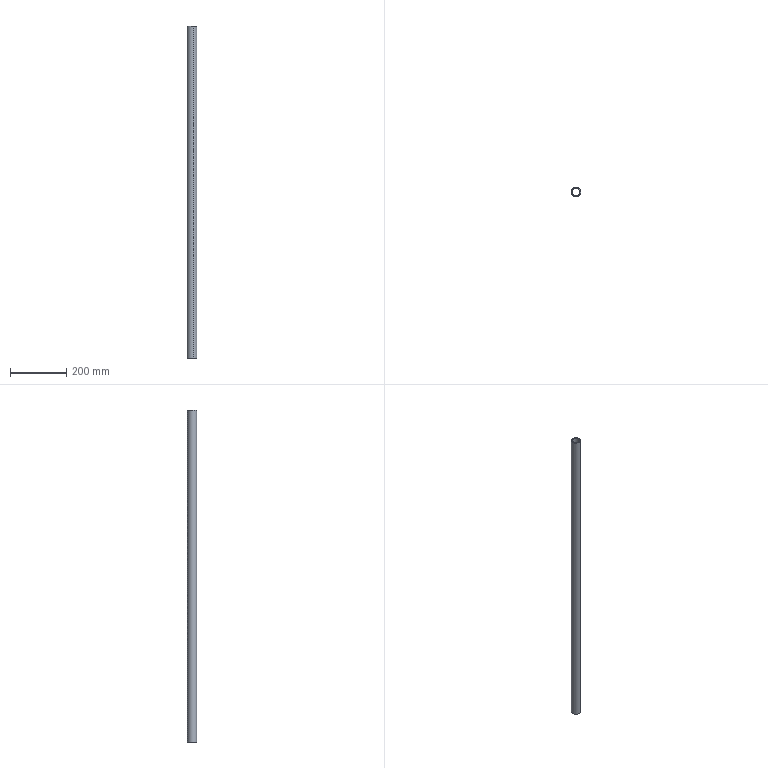Component | SolidWorks | PlatformGuardrail2-10 | 1 solid | 6 faces | box 33.5 x 33.5 x 1180 mm | volume 339198 mm3 | cylinder 4 | plane 2 | commonest cylinder face diameters 27.5 x2 33.5 x2 | material Plain Carbon Steel
build123d program:
from build123d import *

# Parameters (mm, degrees)
SKETCH1_R           = 16.75
SKETCH1_R_2         = 13.75
BOSS_EXTRUDE1_DEPTH = 1180


with BuildPart() as part:
    # Sketch1 → Boss-Extrude1 (new body)
    with BuildSketch(Plane(origin=(0, 0, 0), x_dir=(1, 0, 0), z_dir=(0, 1, 0))):
        with Locations(Location((0, 0, 0), (0, 0, 270))):
            Circle(SKETCH1_R)
        with Locations(Location((0, 0, 0), (0, 0, 270))):
            Circle(SKETCH1_R_2, mode=Mode.SUBTRACT)
    extrude(amount=BOSS_EXTRUDE1_DEPTH)


solid = part.part

# Placed as in the assembly
solid = solid.moved(Location((271.551, 2924.573, 5594.223), (90, 0, 0)))
STEP:
#1=COLOUR_RGB('',0.7922,0.8196,0.9333);
#2=FILL_AREA_STYLE_COLOUR('',#1);
#3=FILL_AREA_STYLE('',(#2));
#4=SURFACE_STYLE_FILL_AREA(#3);
#5=SURFACE_SIDE_STYLE('',(#4));
#6=SURFACE_STYLE_USAGE(.BOTH.,#5);
#7=PRESENTATION_STYLE_ASSIGNMENT((#6));
#8=CARTESIAN_POINT('',(10.52,115.654,266.702));
#9=VERTEX_POINT('',#8);
#10=CARTESIAN_POINT('',(10.862,114.627,266.702));
#11=VERTEX_POINT('',#10);
#12=CARTESIAN_POINT('',(10.691,115.141,266.702));
#13=DIRECTION('',(0.,-0.,1.));
#14=DIRECTION('',(0.3163,-0.9487,0.));
#15=AXIS2_PLACEMENT_3D('',#12,#13,#14);
#16=CIRCLE('',#15,0.5413);
#17=EDGE_CURVE('',#9,#11,#16,.T.);
#18=ORIENTED_EDGE('',*,*,#17,.T.);
#19=CARTESIAN_POINT('',(10.862,114.627,220.245));
#20=VERTEX_POINT('',#19);
#21=CARTESIAN_POINT('',(10.862,114.627,266.702));
#22=DIRECTION('',(-0.,0.,-1.));
#23=VECTOR('',#22,39.37);
#24=LINE('',#21,#23);
#25=EDGE_CURVE('',#11,#20,#24,.T.);
#26=ORIENTED_EDGE('',*,*,#25,.T.);
#27=CARTESIAN_POINT('',(10.52,115.654,220.245));
#28=VERTEX_POINT('',#27);
#29=CARTESIAN_POINT('',(10.691,115.141,220.245));
#30=DIRECTION('',(0.,-0.,1.));
#31=DIRECTION('',(0.3163,-0.9487,0.));
#32=AXIS2_PLACEMENT_3D('',#29,#30,#31);
#33=CIRCLE('',#32,0.5413);
#34=EDGE_CURVE('',#28,#20,#33,.T.);
#35=ORIENTED_EDGE('',*,*,#34,.F.);
#36=CARTESIAN_POINT('',(10.52,115.654,266.702));
#37=DIRECTION('',(-0.,0.,-1.));
#38=VECTOR('',#37,39.37);
#39=LINE('',#36,#38);
#40=EDGE_CURVE('',#9,#28,#39,.T.);
#41=ORIENTED_EDGE('',*,*,#40,.F.);
#42=EDGE_LOOP('',(#18,#26,#35,#41));
#43=FACE_OUTER_BOUND('',#42,.T.);
#44=CARTESIAN_POINT('',(10.691,115.141,266.702));
#45=DIRECTION('',(-0.,0.,-1.));
#46=DIRECTION('',(-0.3163,0.9487,0.));
#47=AXIS2_PLACEMENT_3D('',#44,#45,#46);
#48=CYLINDRICAL_SURFACE('',#47,0.5413);
#49=ADVANCED_FACE('',(#43),#48,.F.);
#50=CARTESIAN_POINT('',(10.9,114.515,266.702));
#51=VERTEX_POINT('',#50);
#52=CARTESIAN_POINT('',(10.482,115.766,266.702));
#53=VERTEX_POINT('',#52);
#54=CARTESIAN_POINT('',(10.691,115.141,266.702));
#55=DIRECTION('',(0.,-0.,1.));
#56=DIRECTION('',(0.3163,-0.9487,0.));
#57=AXIS2_PLACEMENT_3D('',#54,#55,#56);
#58=CIRCLE('',#57,0.6594);
#59=EDGE_CURVE('',#51,#53,#58,.T.);
#60=ORIENTED_EDGE('',*,*,#59,.F.);
#61=CARTESIAN_POINT('',(10.9,114.515,220.245));
#62=VERTEX_POINT('',#61);
#63=CARTESIAN_POINT('',(10.9,114.515,266.702));
#64=DIRECTION('',(-0.,0.,-1.));
#65=VECTOR('',#64,39.37);
#66=LINE('',#63,#65);
#67=EDGE_CURVE('',#51,#62,#66,.T.);
#68=ORIENTED_EDGE('',*,*,#67,.T.);
#69=CARTESIAN_POINT('',(10.482,115.766,220.245));
#70=VERTEX_POINT('',#69);
#71=CARTESIAN_POINT('',(10.691,115.141,220.245));
#72=DIRECTION('',(0.,-0.,1.));
#73=DIRECTION('',(0.3163,-0.9487,0.));
#74=AXIS2_PLACEMENT_3D('',#71,#72,#73);
#75=CIRCLE('',#74,0.6594);
#76=EDGE_CURVE('',#62,#70,#75,.T.);
#77=ORIENTED_EDGE('',*,*,#76,.T.);
#78=CARTESIAN_POINT('',(10.482,115.766,266.702));
#79=DIRECTION('',(-0.,0.,-1.));
#80=VECTOR('',#79,39.37);
#81=LINE('',#78,#80);
#82=EDGE_CURVE('',#53,#70,#81,.T.);
#83=ORIENTED_EDGE('',*,*,#82,.F.);
#84=EDGE_LOOP('',(#60,#68,#77,#83));
#85=FACE_OUTER_BOUND('',#84,.T.);
#86=CARTESIAN_POINT('',(10.691,115.141,266.702));
#87=DIRECTION('',(-0.,0.,-1.));
#88=DIRECTION('',(-0.3163,0.9487,0.));
#89=AXIS2_PLACEMENT_3D('',#86,#87,#88);
#90=CYLINDRICAL_SURFACE('',#89,0.6594);
#91=ADVANCED_FACE('',(#85),#90,.T.);
#92=CARTESIAN_POINT('',(10.691,115.141,266.702));
#93=DIRECTION('',(0.,-0.,1.));
#94=DIRECTION('',(0.3163,-0.9487,0.));
#95=AXIS2_PLACEMENT_3D('',#92,#93,#94);
#96=CIRCLE('',#95,0.6594);
#97=EDGE_CURVE('',#53,#51,#96,.T.);
#98=ORIENTED_EDGE('',*,*,#97,.T.);
#99=ORIENTED_EDGE('',*,*,#59,.T.);
#100=EDGE_LOOP('',(#98,#99));
#101=FACE_OUTER_BOUND('',#100,.T.);
#102=ORIENTED_EDGE('',*,*,#17,.F.);
#103=CARTESIAN_POINT('',(10.691,115.141,266.702));
#104=DIRECTION('',(0.,-0.,1.));
#105=DIRECTION('',(0.3163,-0.9487,0.));
#106=AXIS2_PLACEMENT_3D('',#103,#104,#105);
#107=CIRCLE('',#106,0.5413);
#108=EDGE_CURVE('',#11,#9,#107,.T.);
#109=ORIENTED_EDGE('',*,*,#108,.F.);
#110=EDGE_LOOP('',(#102,#109));
#111=FACE_BOUND('',#110,.T.);
#112=CARTESIAN_POINT('',(10.691,115.141,266.702));
#113=DIRECTION('',(0.,-0.,1.));
#114=DIRECTION('',(0.3163,-0.9487,-0.));
#115=AXIS2_PLACEMENT_3D('',#112,#113,#114);
#116=PLANE('',#115);
#117=ADVANCED_FACE('',(#101,#111),#116,.T.);
#118=CARTESIAN_POINT('',(10.691,115.141,220.245));
#119=DIRECTION('',(0.,-0.,1.));
#120=DIRECTION('',(0.3163,-0.9487,0.));
#121=AXIS2_PLACEMENT_3D('',#118,#119,#120);
#122=CIRCLE('',#121,0.6594);
#123=EDGE_CURVE('',#70,#62,#122,.T.);
#124=ORIENTED_EDGE('',*,*,#123,.F.);
#125=ORIENTED_EDGE('',*,*,#76,.F.);
#126=EDGE_LOOP('',(#124,#125));
#127=FACE_OUTER_BOUND('',#126,.T.);
#128=ORIENTED_EDGE('',*,*,#34,.T.);
#129=CARTESIAN_POINT('',(10.691,115.141,220.245));
#130=DIRECTION('',(0.,-0.,1.));
#131=DIRECTION('',(0.3163,-0.9487,0.));
#132=AXIS2_PLACEMENT_3D('',#129,#130,#131);
#133=CIRCLE('',#132,0.5413);
#134=EDGE_CURVE('',#20,#28,#133,.T.);
#135=ORIENTED_EDGE('',*,*,#134,.T.);
#136=EDGE_LOOP('',(#128,#135));
#137=FACE_BOUND('',#136,.T.);
#138=CARTESIAN_POINT('',(10.691,115.141,220.245));
#139=DIRECTION('',(0.,-0.,1.));
#140=DIRECTION('',(0.3163,-0.9487,-0.));
#141=AXIS2_PLACEMENT_3D('',#138,#139,#140);
#142=PLANE('',#141);
#143=ADVANCED_FACE('',(#127,#137),#142,.F.);
#144=ORIENTED_EDGE('',*,*,#67,.F.);
#145=ORIENTED_EDGE('',*,*,#97,.F.);
#146=ORIENTED_EDGE('',*,*,#82,.T.);
#147=ORIENTED_EDGE('',*,*,#123,.T.);
#148=EDGE_LOOP('',(#144,#145,#146,#147));
#149=FACE_OUTER_BOUND('',#148,.T.);
#150=CARTESIAN_POINT('',(10.691,115.141,266.702));
#151=DIRECTION('',(-0.,0.,-1.));
#152=DIRECTION('',(-0.3163,0.9487,0.));
#153=AXIS2_PLACEMENT_3D('',#150,#151,#152);
#154=CYLINDRICAL_SURFACE('',#153,0.6594);
#155=ADVANCED_FACE('',(#149),#154,.T.);
#156=ORIENTED_EDGE('',*,*,#25,.F.);
#157=ORIENTED_EDGE('',*,*,#108,.T.);
#158=ORIENTED_EDGE('',*,*,#40,.T.);
#159=ORIENTED_EDGE('',*,*,#134,.F.);
#160=EDGE_LOOP('',(#156,#157,#158,#159));
#161=FACE_OUTER_BOUND('',#160,.T.);
#162=CARTESIAN_POINT('',(10.691,115.141,266.702));
#163=DIRECTION('',(-0.,0.,-1.));
#164=DIRECTION('',(-0.3163,0.9487,0.));
#165=AXIS2_PLACEMENT_3D('',#162,#163,#164);
#166=CYLINDRICAL_SURFACE('',#165,0.5413);
#167=ADVANCED_FACE('',(#161),#166,.F.);
#168=CLOSED_SHELL('',(#49,#91,#117,#143,#155,#167));
#169=MANIFOLD_SOLID_BREP('',#168);
#170=STYLED_ITEM('',(#7),#169);
#171=PRESENTATION_LAYER_ASSIGNMENT('','',(#170));
#172=CARTESIAN_POINT('',(0.,0.,0.));
#173=DIRECTION('',(0.,0.,1.));
#174=DIRECTION('',(1.,0.,0.));
#175=AXIS2_PLACEMENT_3D('',#172,#173,#174);
#176=(LENGTH_UNIT()NAMED_UNIT(*)SI_UNIT($,.METRE.));
#177=LENGTH_MEASURE_WITH_UNIT(LENGTH_MEASURE(0.0254),#176);
#178=DIMENSIONAL_EXPONENTS(1.,0.,0.,0.,0.,0.,0.);
#179=(CONVERSION_BASED_UNIT('',#177)LENGTH_UNIT()NAMED_UNIT(#178));
#180=UNCERTAINTY_MEASURE_WITH_UNIT(LENGTH_MEASURE(0.00001),#179,'','');
#181=(NAMED_UNIT(*)PLANE_ANGLE_UNIT()SI_UNIT($,.RADIAN.));
#182=(NAMED_UNIT(*)SI_UNIT($,.STERADIAN.)SOLID_ANGLE_UNIT());
#183=(GEOMETRIC_REPRESENTATION_CONTEXT(3)GLOBAL_UNCERTAINTY_ASSIGNED_CONTEXT((#180))GLOBAL_UNIT_ASSIGNED_CONTEXT((#179,#181,#182))REPRESENTATION_CONTEXT('',''));
#184=ADVANCED_BREP_SHAPE_REPRESENTATION('',(#169,#175),#183);
#185=(LENGTH_UNIT()NAMED_UNIT(*)SI_UNIT($,.METRE.));
#186=LENGTH_MEASURE_WITH_UNIT(LENGTH_MEASURE(0.0254),#185);
#187=DIMENSIONAL_EXPONENTS(1.,0.,0.,0.,0.,0.,0.);
#188=(CONVERSION_BASED_UNIT('',#186)LENGTH_UNIT()NAMED_UNIT(#187));
#189=UNCERTAINTY_MEASURE_WITH_UNIT(LENGTH_MEASURE(0.00001),#188,'','');
#190=(NAMED_UNIT(*)PLANE_ANGLE_UNIT()SI_UNIT($,.RADIAN.));
#191=(NAMED_UNIT(*)SI_UNIT($,.STERADIAN.)SOLID_ANGLE_UNIT());
#192=(GEOMETRIC_REPRESENTATION_CONTEXT(3)GLOBAL_UNCERTAINTY_ASSIGNED_CONTEXT((#189))GLOBAL_UNIT_ASSIGNED_CONTEXT((#188,#190,#191))REPRESENTATION_CONTEXT('',''));
#193=MECHANICAL_DESIGN_GEOMETRIC_PRESENTATION_REPRESENTATION('',(#170),#192);